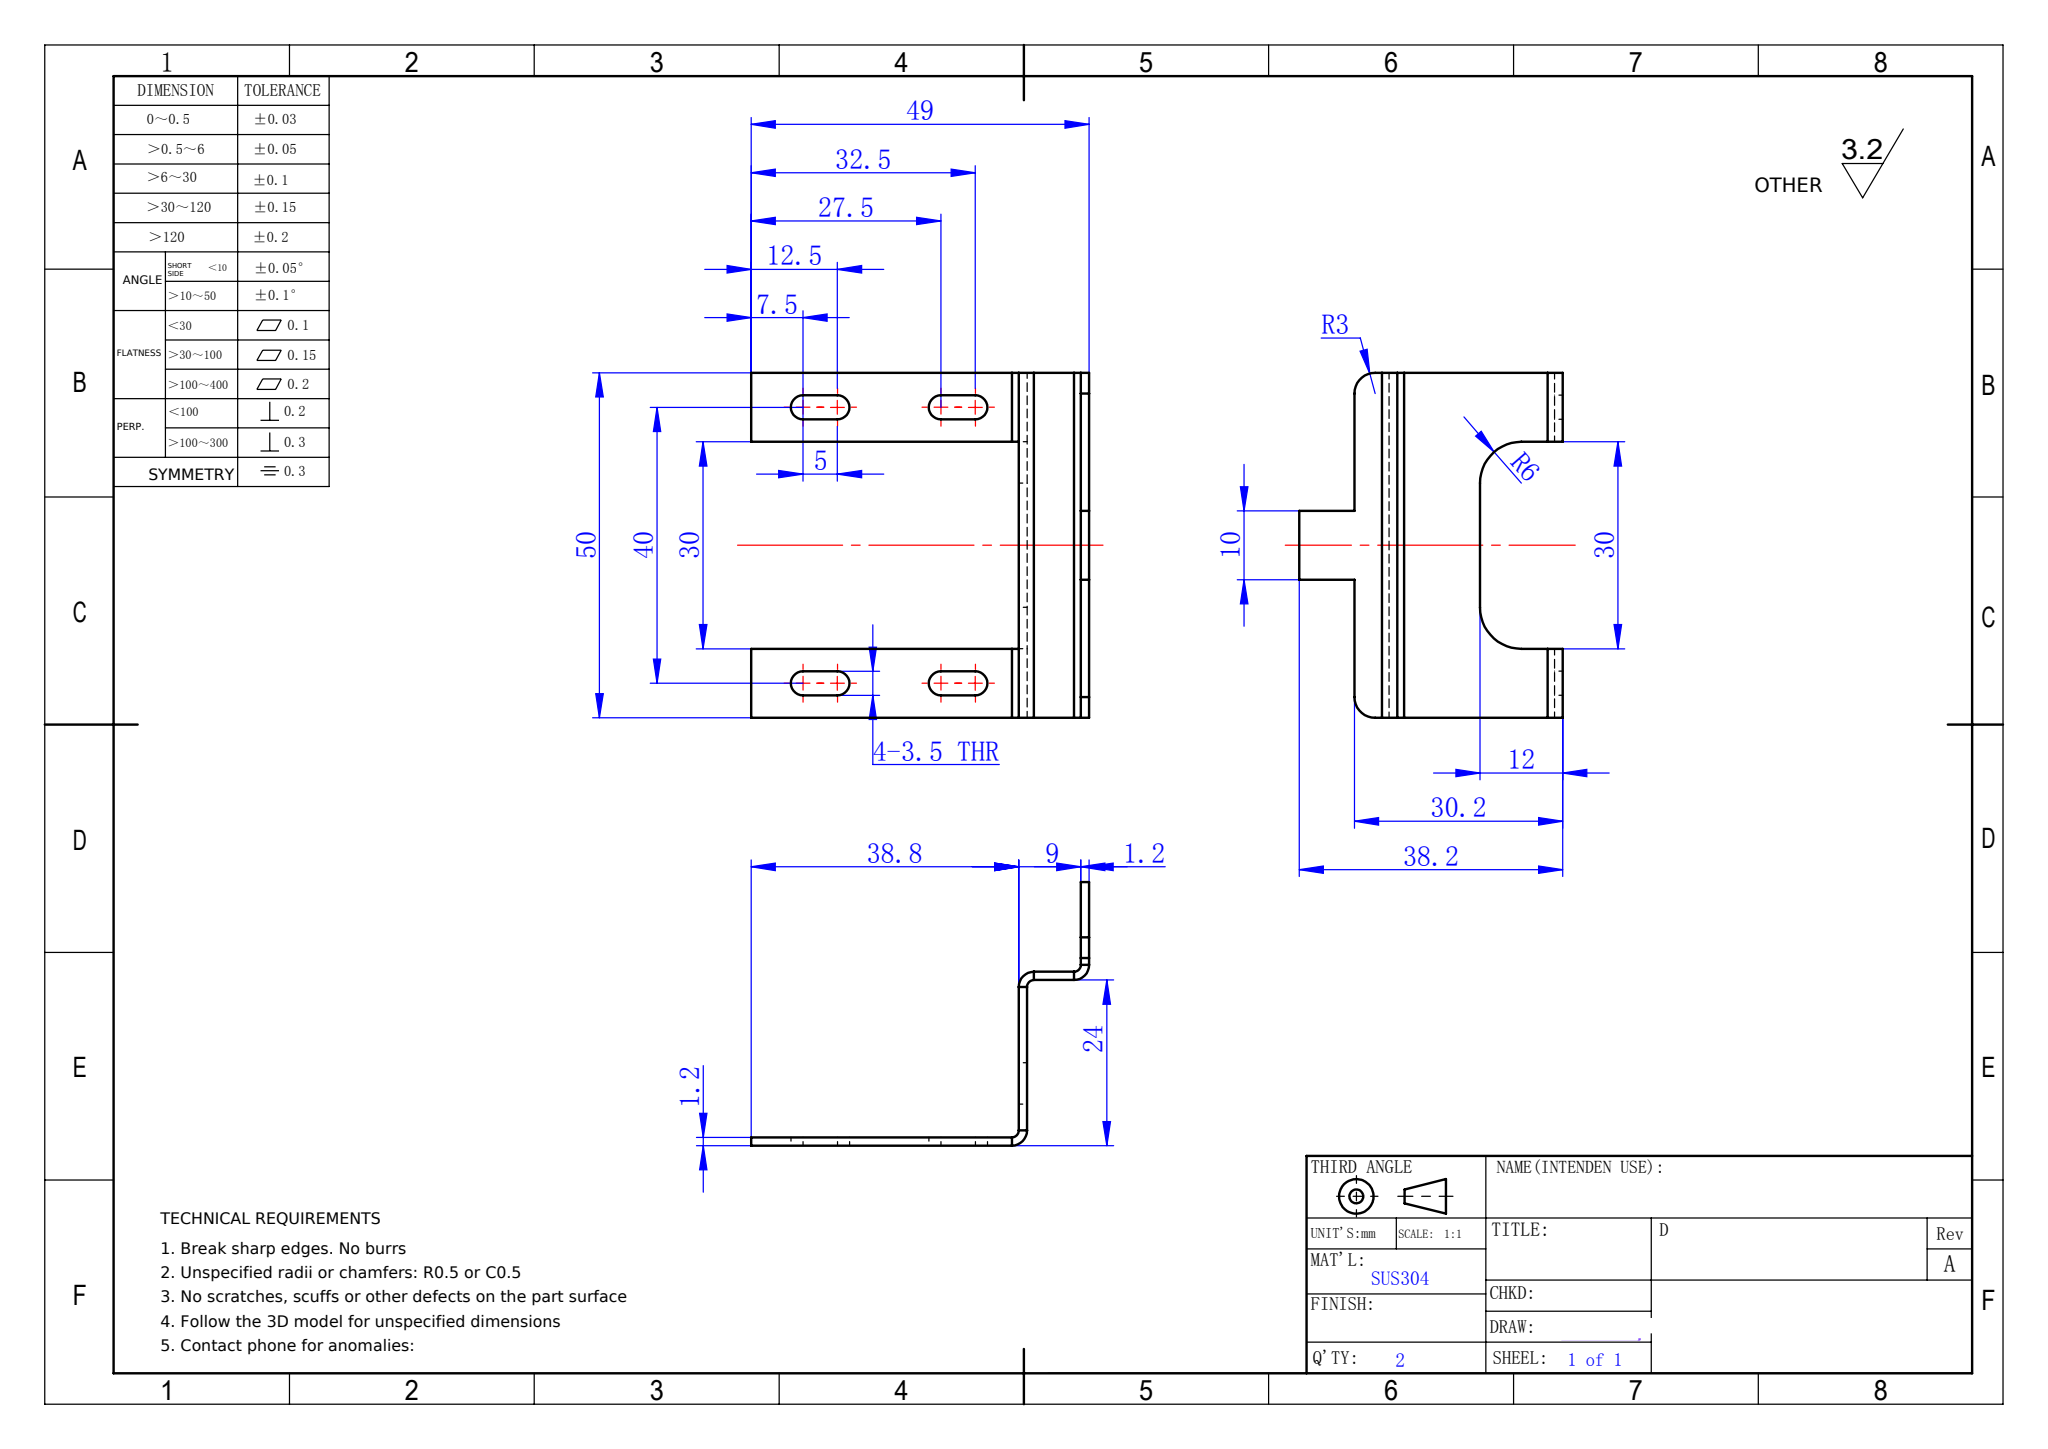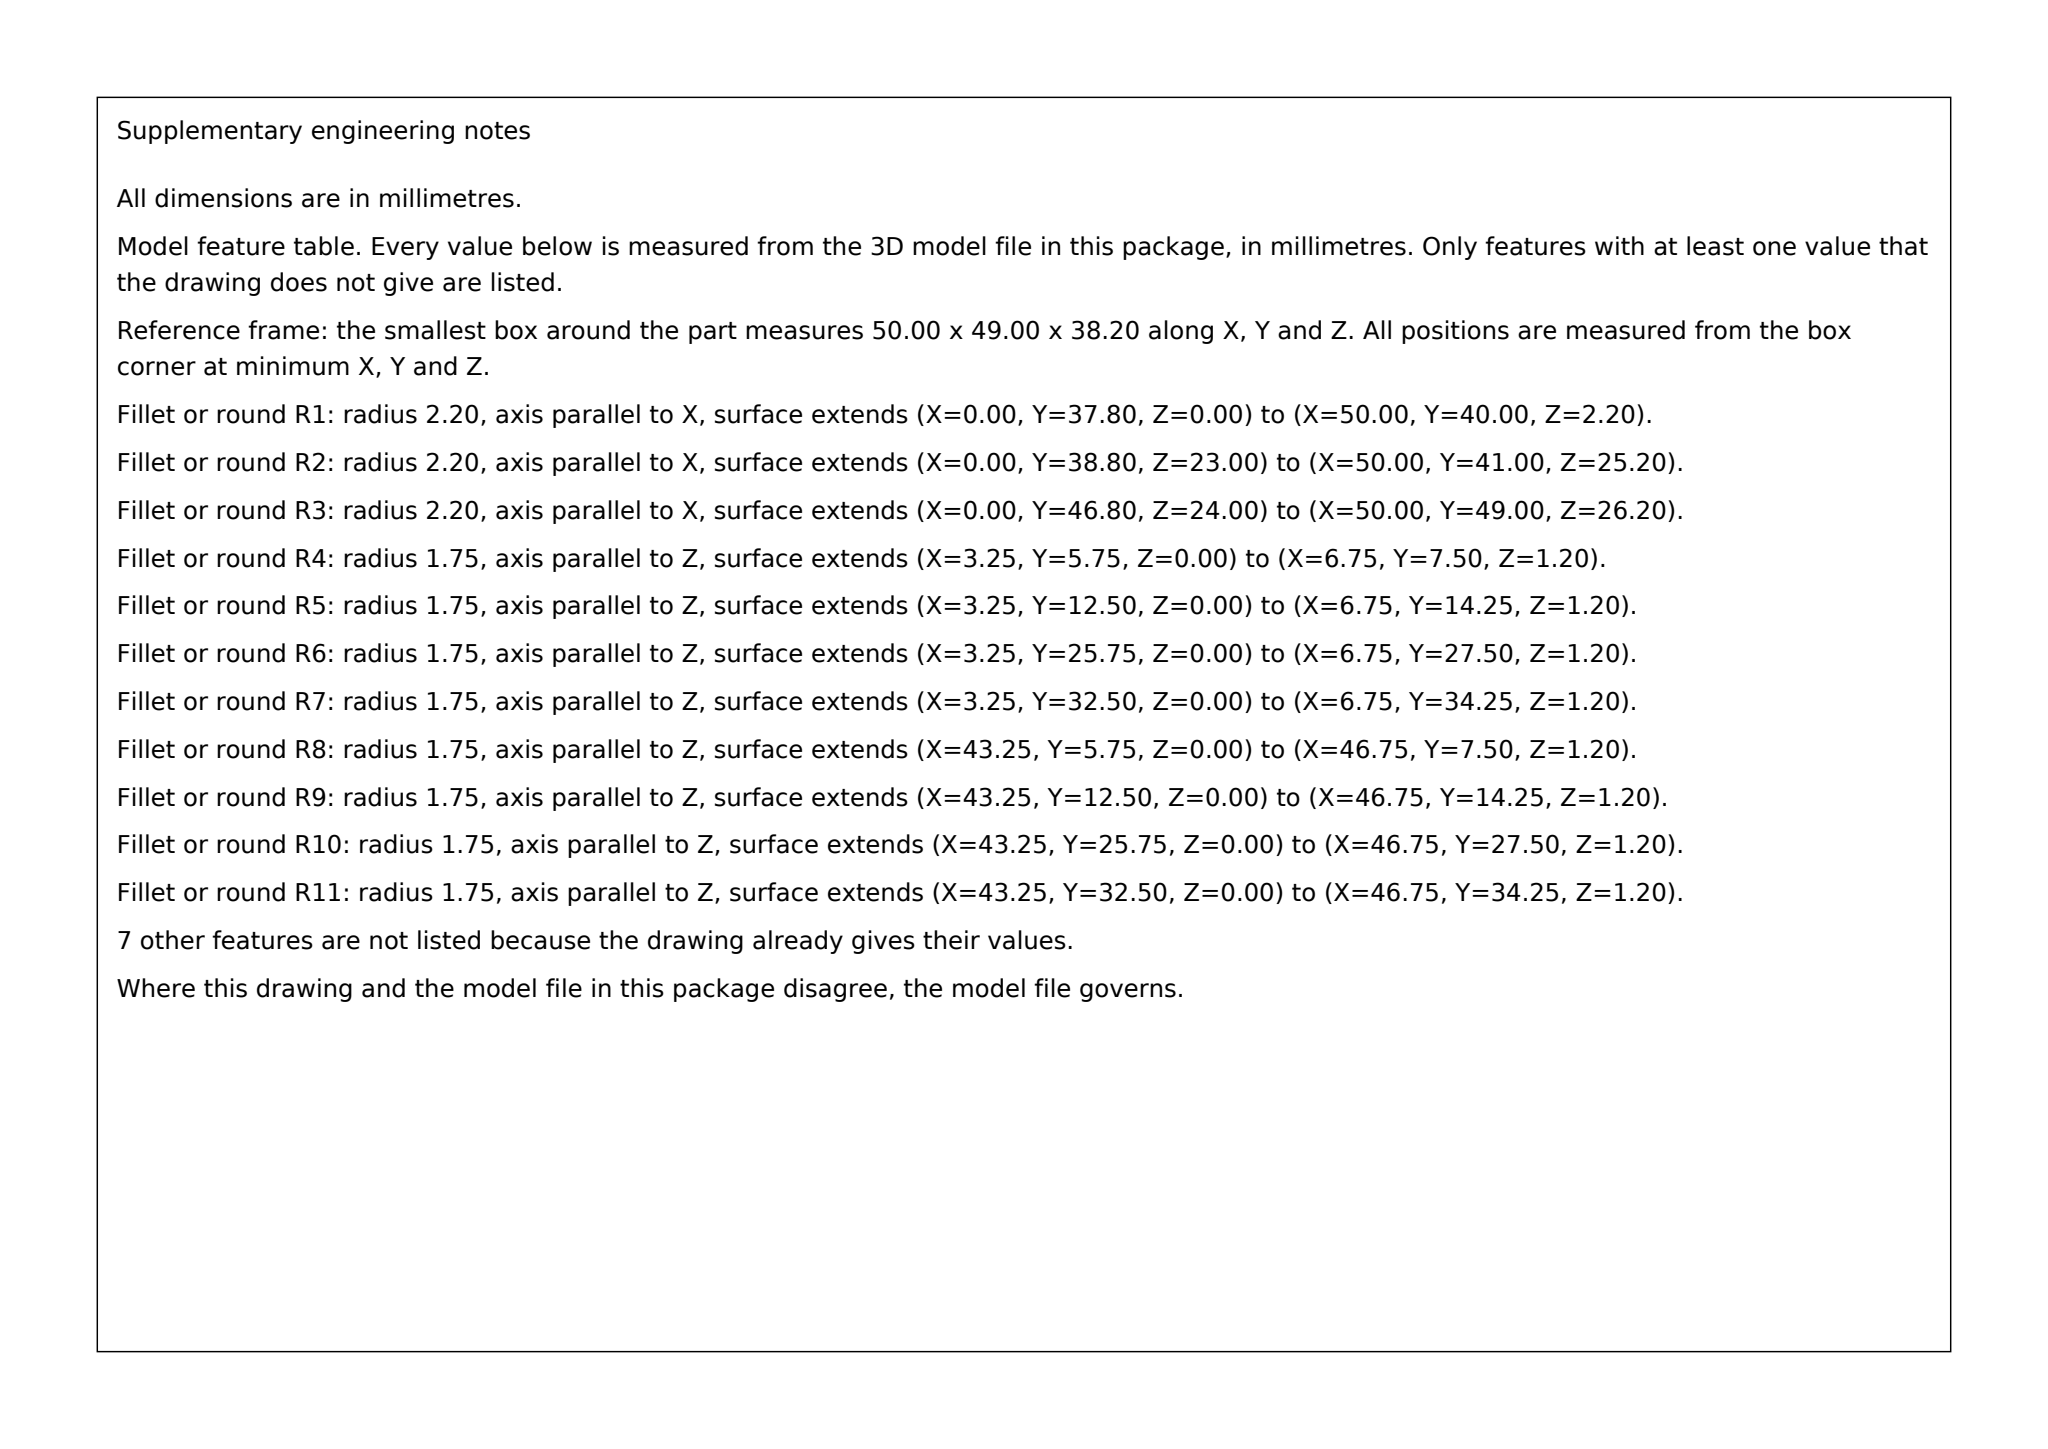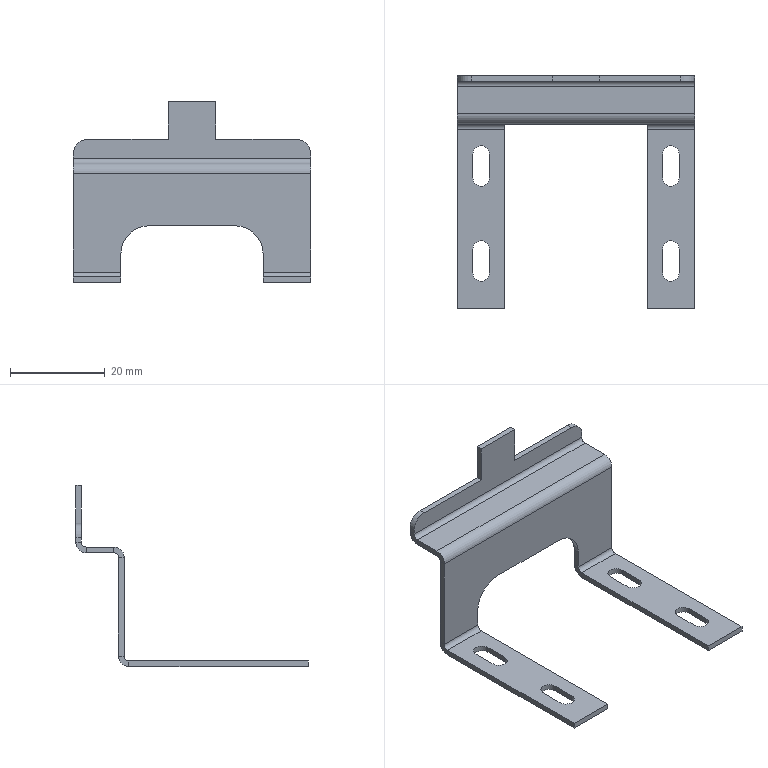Part | SolidWorks | mm | 1 solid | 66 faces | box 50 x 49 x 38.2 mm | volume 2732 mm3 | plane 46 | cylinder 20 | commonest cylinder face diameters 3.5 x8 4.4 x4 2 x4 12 x2 6 x2